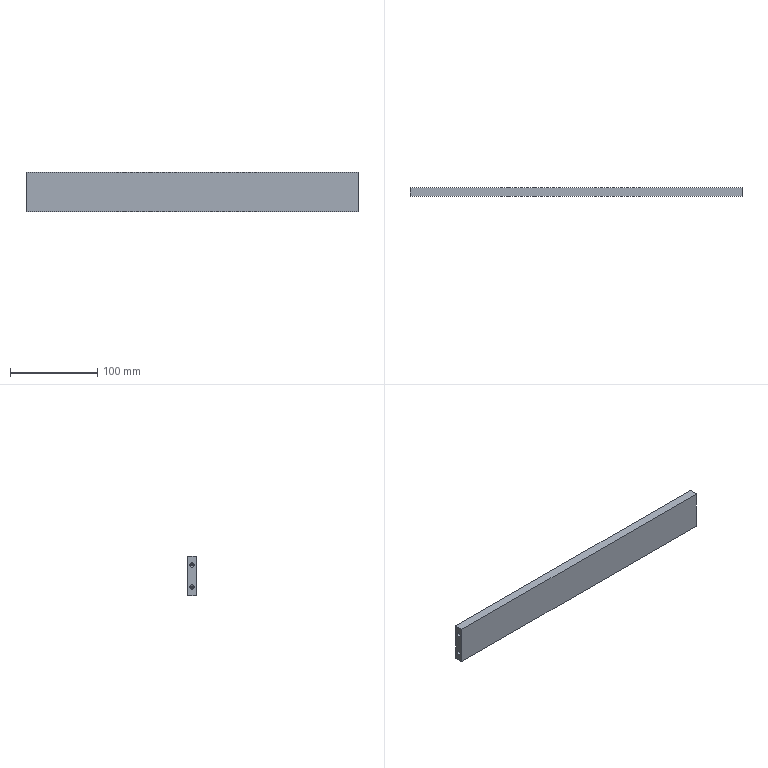Component | SolidWorks | 01-08MarkingMachineDrumConnectingPlate2-1 | 1 solid | 22 faces | box 380 x 10 x 45 mm | volume 169783 mm3 | cylinder 8 | cone 8 | plane 6 | commonest cylinder face diameters 5 x8 | material A3 Steel
build123d program:
from build123d import *

# Parameters (mm, degrees)
SKETCH1_W                  = 380
SKETCH1_H                  = 45
BOSS_EXTRUDE1_DEPTH        = 5
M6_TAPPED_HOLE1_AT_2_COUNT = 2
M6_TAPPED_HOLE1_AT_2_PITCH = 25


with BuildPart() as part:
    # Sketch1 → Boss-Extrude1 (new, symmetric)
    with BuildSketch(Plane.XY):
        Rectangle(SKETCH1_W, SKETCH1_H)
    extrude(amount=BOSS_EXTRUDE1_DEPTH, both=True)

    # Sketch4 → M6 Tapped Hole1 (revolve, cut)
    with BuildSketch(Plane(origin=(190, 12.5, 0), x_dir=(0, 0, -1), z_dir=(0, 1, 0))):
        Polygon((0, 0), (0, 16.502), (2.5, 15), (2.5, 0), align=None)
    m6_tapped_hole1 = revolve(axis=Axis((196.35, 12.5, 0), (-1, 0, 0)), mode=Mode.SUBTRACT)

    # M6 Tapped Hole1 at 2: M6 Tapped Hole1 ×2
    with Locations(*[(0, -i * M6_TAPPED_HOLE1_AT_2_PITCH, 0) for i in range(1, M6_TAPPED_HOLE1_AT_2_COUNT)]):
        add(m6_tapped_hole1, mode=Mode.SUBTRACT)

    # Mirror1: M6 Tapped Hole1 across plane
    add(m6_tapped_hole1.mirror(Plane(origin=(0, 0, 0), x_dir=(0, 0, 1), z_dir=(1, 0, 0))), mode=Mode.SUBTRACT)

    # Mirror1 copy 1 sketch → Mirror1 copy 1 (revolve, cut)
    with BuildSketch(Plane(origin=(-190, -12.5, 0), x_dir=(0, 0, -1), z_dir=(0, 1, 0))):
        Polygon((0, 0), (0, -16.502), (2.5, -15), (2.5, 0), align=None)
    revolve(axis=Axis((-196.35, -12.5, 0), (-1, 0, 0)), mode=Mode.SUBTRACT)


solid = part.part

# Placed as in the assembly
solid = solid.moved(Location((-256.91, 2.41, -167.5), (90, 0, 0)))
STEP:
#1=COLOUR_RGB('',0.7922,0.8196,0.9333);
#2=FILL_AREA_STYLE_COLOUR('',#1);
#3=FILL_AREA_STYLE('',(#2));
#4=SURFACE_STYLE_FILL_AREA(#3);
#5=SURFACE_SIDE_STYLE('',(#4));
#6=SURFACE_STYLE_USAGE(.BOTH.,#5);
#7=PRESENTATION_STYLE_ASSIGNMENT((#6));
#8=CARTESIAN_POINT('',(-17.004,0.1933,-6.102));
#9=VERTEX_POINT('',#8);
#10=CARTESIAN_POINT('',(-17.004,-0.003525,-6.102));
#11=VERTEX_POINT('',#10);
#12=CARTESIAN_POINT('',(-17.004,0.0949,-6.102));
#13=DIRECTION('',(-1.,0.,0.));
#14=DIRECTION('',(0.,-1.,0.));
#15=AXIS2_PLACEMENT_3D('',#12,#13,#14);
#16=CIRCLE('',#15,0.09843);
#17=EDGE_CURVE('',#9,#11,#16,.T.);
#18=ORIENTED_EDGE('',*,*,#17,.F.);
#19=CARTESIAN_POINT('',(-17.595,0.1933,-6.102));
#20=VERTEX_POINT('',#19);
#21=CARTESIAN_POINT('',(-17.595,0.1933,-6.102));
#22=DIRECTION('',(-1.,0.,0.));
#23=VECTOR('',#22,39.37);
#24=LINE('',#21,#23);
#25=EDGE_CURVE('',#9,#20,#24,.T.);
#26=ORIENTED_EDGE('',*,*,#25,.T.);
#27=CARTESIAN_POINT('',(-17.595,-0.003525,-6.102));
#28=VERTEX_POINT('',#27);
#29=CARTESIAN_POINT('',(-17.595,0.0949,-6.102));
#30=DIRECTION('',(-1.,0.,0.));
#31=DIRECTION('',(0.,-1.,0.));
#32=AXIS2_PLACEMENT_3D('',#29,#30,#31);
#33=CIRCLE('',#32,0.09843);
#34=EDGE_CURVE('',#20,#28,#33,.T.);
#35=ORIENTED_EDGE('',*,*,#34,.T.);
#36=CARTESIAN_POINT('',(-17.595,-0.003525,-6.102));
#37=DIRECTION('',(-1.,0.,0.));
#38=VECTOR('',#37,39.37);
#39=LINE('',#36,#38);
#40=EDGE_CURVE('',#11,#28,#39,.T.);
#41=ORIENTED_EDGE('',*,*,#40,.F.);
#42=EDGE_LOOP('',(#18,#26,#35,#41));
#43=FACE_OUTER_BOUND('',#42,.T.);
#44=CARTESIAN_POINT('',(-17.595,0.0949,-6.102));
#45=DIRECTION('',(-1.,0.,0.));
#46=DIRECTION('',(0.,-1.,0.));
#47=AXIS2_PLACEMENT_3D('',#44,#45,#46);
#48=CYLINDRICAL_SURFACE('',#47,0.09843);
#49=ADVANCED_FACE('',(#43),#48,.F.);
#50=CARTESIAN_POINT('',(-16.945,0.0949,-6.102));
#51=VERTEX_POINT('',#50);
#52=CARTESIAN_POINT('',(-17.004,-0.003525,-6.102));
#53=DIRECTION('',(-0.515,-0.8572,-0.));
#54=VECTOR('',#53,39.37);
#55=LINE('',#52,#54);
#56=EDGE_CURVE('',#51,#11,#55,.T.);
#57=ORIENTED_EDGE('',*,*,#56,.F.);
#58=CARTESIAN_POINT('',(-17.004,0.1933,-6.102));
#59=DIRECTION('',(-0.515,0.8572,0.));
#60=VECTOR('',#59,39.37);
#61=LINE('',#58,#60);
#62=EDGE_CURVE('',#51,#9,#61,.T.);
#63=ORIENTED_EDGE('',*,*,#62,.T.);
#64=ORIENTED_EDGE('',*,*,#17,.T.);
#65=EDGE_LOOP('',(#57,#63,#64));
#66=FACE_OUTER_BOUND('',#65,.T.);
#67=CARTESIAN_POINT('',(-17.004,0.0949,-6.102));
#68=DIRECTION('',(-1.,0.,0.));
#69=DIRECTION('',(0.,-1.,0.));
#70=AXIS2_PLACEMENT_3D('',#67,#68,#69);
#71=CONICAL_SURFACE('',#70,0.09843,1.03);
#72=ADVANCED_FACE('',(#66),#71,.F.);
#73=CARTESIAN_POINT('',(-17.004,0.1933,-7.087));
#74=VERTEX_POINT('',#73);
#75=CARTESIAN_POINT('',(-17.004,-0.003525,-7.087));
#76=VERTEX_POINT('',#75);
#77=CARTESIAN_POINT('',(-17.004,0.0949,-7.087));
#78=DIRECTION('',(-1.,0.,0.));
#79=DIRECTION('',(0.,-1.,0.));
#80=AXIS2_PLACEMENT_3D('',#77,#78,#79);
#81=CIRCLE('',#80,0.09843);
#82=EDGE_CURVE('',#74,#76,#81,.T.);
#83=ORIENTED_EDGE('',*,*,#82,.F.);
#84=CARTESIAN_POINT('',(-17.595,0.1933,-7.087));
#85=VERTEX_POINT('',#84);
#86=CARTESIAN_POINT('',(-17.595,0.1933,-7.087));
#87=DIRECTION('',(-1.,0.,0.));
#88=VECTOR('',#87,39.37);
#89=LINE('',#86,#88);
#90=EDGE_CURVE('',#74,#85,#89,.T.);
#91=ORIENTED_EDGE('',*,*,#90,.T.);
#92=CARTESIAN_POINT('',(-17.595,-0.003525,-7.087));
#93=VERTEX_POINT('',#92);
#94=CARTESIAN_POINT('',(-17.595,0.0949,-7.087));
#95=DIRECTION('',(-1.,0.,0.));
#96=DIRECTION('',(0.,-1.,0.));
#97=AXIS2_PLACEMENT_3D('',#94,#95,#96);
#98=CIRCLE('',#97,0.09843);
#99=EDGE_CURVE('',#85,#93,#98,.T.);
#100=ORIENTED_EDGE('',*,*,#99,.T.);
#101=CARTESIAN_POINT('',(-17.595,-0.003525,-7.087));
#102=DIRECTION('',(-1.,0.,0.));
#103=VECTOR('',#102,39.37);
#104=LINE('',#101,#103);
#105=EDGE_CURVE('',#76,#93,#104,.T.);
#106=ORIENTED_EDGE('',*,*,#105,.F.);
#107=EDGE_LOOP('',(#83,#91,#100,#106));
#108=FACE_OUTER_BOUND('',#107,.T.);
#109=CARTESIAN_POINT('',(-17.595,0.0949,-7.087));
#110=DIRECTION('',(-1.,0.,0.));
#111=DIRECTION('',(0.,-1.,0.));
#112=AXIS2_PLACEMENT_3D('',#109,#110,#111);
#113=CYLINDRICAL_SURFACE('',#112,0.09843);
#114=ADVANCED_FACE('',(#108),#113,.F.);
#115=CARTESIAN_POINT('',(-16.945,0.0949,-7.087));
#116=VERTEX_POINT('',#115);
#117=CARTESIAN_POINT('',(-17.004,-0.003525,-7.087));
#118=DIRECTION('',(-0.515,-0.8572,-0.));
#119=VECTOR('',#118,39.37);
#120=LINE('',#117,#119);
#121=EDGE_CURVE('',#116,#76,#120,.T.);
#122=ORIENTED_EDGE('',*,*,#121,.F.);
#123=CARTESIAN_POINT('',(-17.004,0.1933,-7.087));
#124=DIRECTION('',(-0.515,0.8572,0.));
#125=VECTOR('',#124,39.37);
#126=LINE('',#123,#125);
#127=EDGE_CURVE('',#116,#74,#126,.T.);
#128=ORIENTED_EDGE('',*,*,#127,.T.);
#129=ORIENTED_EDGE('',*,*,#82,.T.);
#130=EDGE_LOOP('',(#122,#128,#129));
#131=FACE_OUTER_BOUND('',#130,.T.);
#132=CARTESIAN_POINT('',(-17.004,0.0949,-7.087));
#133=DIRECTION('',(-1.,0.,0.));
#134=DIRECTION('',(0.,-1.,0.));
#135=AXIS2_PLACEMENT_3D('',#132,#133,#134);
#136=CONICAL_SURFACE('',#135,0.09843,1.03);
#137=ADVANCED_FACE('',(#131),#136,.F.);
#138=CARTESIAN_POINT('',(-3.225,-0.003525,-6.102));
#139=VERTEX_POINT('',#138);
#140=CARTESIAN_POINT('',(-3.225,0.1933,-6.102));
#141=VERTEX_POINT('',#140);
#142=CARTESIAN_POINT('',(-3.225,0.0949,-6.102));
#143=DIRECTION('',(1.,-0.,-0.));
#144=DIRECTION('',(0.,1.,0.));
#145=AXIS2_PLACEMENT_3D('',#142,#143,#144);
#146=CIRCLE('',#145,0.09843);
#147=EDGE_CURVE('',#139,#141,#146,.T.);
#148=ORIENTED_EDGE('',*,*,#147,.F.);
#149=CARTESIAN_POINT('',(-2.634,-0.003525,-6.102));
#150=VERTEX_POINT('',#149);
#151=CARTESIAN_POINT('',(-2.634,-0.003525,-6.102));
#152=DIRECTION('',(1.,-0.,-0.));
#153=VECTOR('',#152,39.37);
#154=LINE('',#151,#153);
#155=EDGE_CURVE('',#139,#150,#154,.T.);
#156=ORIENTED_EDGE('',*,*,#155,.T.);
#157=CARTESIAN_POINT('',(-2.634,0.1933,-6.102));
#158=VERTEX_POINT('',#157);
#159=CARTESIAN_POINT('',(-2.634,0.0949,-6.102));
#160=DIRECTION('',(1.,-0.,-0.));
#161=DIRECTION('',(0.,1.,0.));
#162=AXIS2_PLACEMENT_3D('',#159,#160,#161);
#163=CIRCLE('',#162,0.09843);
#164=EDGE_CURVE('',#150,#158,#163,.T.);
#165=ORIENTED_EDGE('',*,*,#164,.T.);
#166=CARTESIAN_POINT('',(-2.634,0.1933,-6.102));
#167=DIRECTION('',(1.,-0.,-0.));
#168=VECTOR('',#167,39.37);
#169=LINE('',#166,#168);
#170=EDGE_CURVE('',#141,#158,#169,.T.);
#171=ORIENTED_EDGE('',*,*,#170,.F.);
#172=EDGE_LOOP('',(#148,#156,#165,#171));
#173=FACE_OUTER_BOUND('',#172,.T.);
#174=CARTESIAN_POINT('',(-2.634,0.0949,-6.102));
#175=DIRECTION('',(1.,-0.,-0.));
#176=DIRECTION('',(0.,1.,0.));
#177=AXIS2_PLACEMENT_3D('',#174,#175,#176);
#178=CYLINDRICAL_SURFACE('',#177,0.09843);
#179=ADVANCED_FACE('',(#173),#178,.F.);
#180=CARTESIAN_POINT('',(-3.284,0.0949,-6.102));
#181=VERTEX_POINT('',#180);
#182=CARTESIAN_POINT('',(-3.225,0.1933,-6.102));
#183=DIRECTION('',(0.515,0.8572,0.));
#184=VECTOR('',#183,39.37);
#185=LINE('',#182,#184);
#186=EDGE_CURVE('',#181,#141,#185,.T.);
#187=ORIENTED_EDGE('',*,*,#186,.F.);
#188=CARTESIAN_POINT('',(-3.225,-0.003525,-6.102));
#189=DIRECTION('',(0.515,-0.8572,0.));
#190=VECTOR('',#189,39.37);
#191=LINE('',#188,#190);
#192=EDGE_CURVE('',#181,#139,#191,.T.);
#193=ORIENTED_EDGE('',*,*,#192,.T.);
#194=ORIENTED_EDGE('',*,*,#147,.T.);
#195=EDGE_LOOP('',(#187,#193,#194));
#196=FACE_OUTER_BOUND('',#195,.T.);
#197=CARTESIAN_POINT('',(-3.225,0.0949,-6.102));
#198=DIRECTION('',(1.,-0.,-0.));
#199=DIRECTION('',(0.,1.,0.));
#200=AXIS2_PLACEMENT_3D('',#197,#198,#199);
#201=CONICAL_SURFACE('',#200,0.09843,1.03);
#202=ADVANCED_FACE('',(#196),#201,.F.);
#203=CARTESIAN_POINT('',(-3.225,-0.003525,-7.087));
#204=VERTEX_POINT('',#203);
#205=CARTESIAN_POINT('',(-3.225,0.1933,-7.087));
#206=VERTEX_POINT('',#205);
#207=CARTESIAN_POINT('',(-3.225,0.0949,-7.087));
#208=DIRECTION('',(1.,-0.,-0.));
#209=DIRECTION('',(0.,1.,0.));
#210=AXIS2_PLACEMENT_3D('',#207,#208,#209);
#211=CIRCLE('',#210,0.09843);
#212=EDGE_CURVE('',#204,#206,#211,.T.);
#213=ORIENTED_EDGE('',*,*,#212,.F.);
#214=CARTESIAN_POINT('',(-2.634,-0.003525,-7.087));
#215=VERTEX_POINT('',#214);
#216=CARTESIAN_POINT('',(-2.634,-0.003525,-7.087));
#217=DIRECTION('',(1.,-0.,-0.));
#218=VECTOR('',#217,39.37);
#219=LINE('',#216,#218);
#220=EDGE_CURVE('',#204,#215,#219,.T.);
#221=ORIENTED_EDGE('',*,*,#220,.T.);
#222=CARTESIAN_POINT('',(-2.634,0.1933,-7.087));
#223=VERTEX_POINT('',#222);
#224=CARTESIAN_POINT('',(-2.634,0.0949,-7.087));
#225=DIRECTION('',(1.,-0.,-0.));
#226=DIRECTION('',(0.,1.,0.));
#227=AXIS2_PLACEMENT_3D('',#224,#225,#226);
#228=CIRCLE('',#227,0.09843);
#229=EDGE_CURVE('',#215,#223,#228,.T.);
#230=ORIENTED_EDGE('',*,*,#229,.T.);
#231=CARTESIAN_POINT('',(-2.634,0.1933,-7.087));
#232=DIRECTION('',(1.,-0.,-0.));
#233=VECTOR('',#232,39.37);
#234=LINE('',#231,#233);
#235=EDGE_CURVE('',#206,#223,#234,.T.);
#236=ORIENTED_EDGE('',*,*,#235,.F.);
#237=EDGE_LOOP('',(#213,#221,#230,#236));
#238=FACE_OUTER_BOUND('',#237,.T.);
#239=CARTESIAN_POINT('',(-2.634,0.0949,-7.087));
#240=DIRECTION('',(1.,-0.,-0.));
#241=DIRECTION('',(0.,1.,0.));
#242=AXIS2_PLACEMENT_3D('',#239,#240,#241);
#243=CYLINDRICAL_SURFACE('',#242,0.09843);
#244=ADVANCED_FACE('',(#238),#243,.F.);
#245=CARTESIAN_POINT('',(-3.284,0.0949,-7.087));
#246=VERTEX_POINT('',#245);
#247=CARTESIAN_POINT('',(-3.225,0.1933,-7.087));
#248=DIRECTION('',(0.515,0.8572,0.));
#249=VECTOR('',#248,39.37);
#250=LINE('',#247,#249);
#251=EDGE_CURVE('',#246,#206,#250,.T.);
#252=ORIENTED_EDGE('',*,*,#251,.F.);
#253=CARTESIAN_POINT('',(-3.225,-0.003525,-7.087));
#254=DIRECTION('',(0.515,-0.8572,0.));
#255=VECTOR('',#254,39.37);
#256=LINE('',#253,#255);
#257=EDGE_CURVE('',#246,#204,#256,.T.);
#258=ORIENTED_EDGE('',*,*,#257,.T.);
#259=ORIENTED_EDGE('',*,*,#212,.T.);
#260=EDGE_LOOP('',(#252,#258,#259));
#261=FACE_OUTER_BOUND('',#260,.T.);
#262=CARTESIAN_POINT('',(-3.225,0.0949,-7.087));
#263=DIRECTION('',(1.,-0.,-0.));
#264=DIRECTION('',(0.,1.,0.));
#265=AXIS2_PLACEMENT_3D('',#262,#263,#264);
#266=CONICAL_SURFACE('',#265,0.09843,1.03);
#267=ADVANCED_FACE('',(#261),#266,.F.);
#268=CARTESIAN_POINT('',(-17.595,0.0949,-7.087));
#269=DIRECTION('',(-1.,0.,0.));
#270=DIRECTION('',(0.,-1.,0.));
#271=AXIS2_PLACEMENT_3D('',#268,#269,#270);
#272=CIRCLE('',#271,0.09843);
#273=EDGE_CURVE('',#93,#85,#272,.T.);
#274=ORIENTED_EDGE('',*,*,#273,.F.);
#275=ORIENTED_EDGE('',*,*,#99,.F.);
#276=EDGE_LOOP('',(#274,#275));
#277=FACE_BOUND('',#276,.T.);
#278=CARTESIAN_POINT('',(-17.595,0.2918,-5.709));
#279=VERTEX_POINT('',#278);
#280=CARTESIAN_POINT('',(-17.595,0.2918,-7.48));
#281=VERTEX_POINT('',#280);
#282=CARTESIAN_POINT('',(-17.595,0.2918,-7.48));
#283=DIRECTION('',(-0.,0.,-1.));
#284=VECTOR('',#283,39.37);
#285=LINE('',#282,#284);
#286=EDGE_CURVE('',#279,#281,#285,.T.);
#287=ORIENTED_EDGE('',*,*,#286,.T.);
#288=CARTESIAN_POINT('',(-17.595,-0.102,-7.48));
#289=VERTEX_POINT('',#288);
#290=CARTESIAN_POINT('',(-17.595,-0.102,-7.48));
#291=DIRECTION('',(0.,1.,0.));
#292=VECTOR('',#291,39.37);
#293=LINE('',#290,#292);
#294=EDGE_CURVE('',#289,#281,#293,.T.);
#295=ORIENTED_EDGE('',*,*,#294,.F.);
#296=CARTESIAN_POINT('',(-17.595,-0.102,-5.709));
#297=VERTEX_POINT('',#296);
#298=CARTESIAN_POINT('',(-17.595,-0.102,-7.48));
#299=DIRECTION('',(-0.,0.,-1.));
#300=VECTOR('',#299,39.37);
#301=LINE('',#298,#300);
#302=EDGE_CURVE('',#297,#289,#301,.T.);
#303=ORIENTED_EDGE('',*,*,#302,.F.);
#304=CARTESIAN_POINT('',(-17.595,-0.102,-5.709));
#305=DIRECTION('',(0.,1.,0.));
#306=VECTOR('',#305,39.37);
#307=LINE('',#304,#306);
#308=EDGE_CURVE('',#297,#279,#307,.T.);
#309=ORIENTED_EDGE('',*,*,#308,.T.);
#310=EDGE_LOOP('',(#287,#295,#303,#309));
#311=FACE_OUTER_BOUND('',#310,.T.);
#312=CARTESIAN_POINT('',(-17.595,0.0949,-6.102));
#313=DIRECTION('',(-1.,0.,0.));
#314=DIRECTION('',(0.,-1.,0.));
#315=AXIS2_PLACEMENT_3D('',#312,#313,#314);
#316=CIRCLE('',#315,0.09843);
#317=EDGE_CURVE('',#28,#20,#316,.T.);
#318=ORIENTED_EDGE('',*,*,#317,.F.);
#319=ORIENTED_EDGE('',*,*,#34,.F.);
#320=EDGE_LOOP('',(#318,#319));
#321=FACE_BOUND('',#320,.T.);
#322=CARTESIAN_POINT('',(-17.595,-0.102,-7.48));
#323=DIRECTION('',(1.,-0.,-0.));
#324=DIRECTION('',(0.,1.,0.));
#325=AXIS2_PLACEMENT_3D('',#322,#323,#324);
#326=PLANE('',#325);
#327=ADVANCED_FACE('',(#277,#311,#321),#326,.F.);
#328=CARTESIAN_POINT('',(-2.634,0.0949,-7.087));
#329=DIRECTION('',(1.,-0.,-0.));
#330=DIRECTION('',(0.,1.,0.));
#331=AXIS2_PLACEMENT_3D('',#328,#329,#330);
#332=CIRCLE('',#331,0.09843);
#333=EDGE_CURVE('',#223,#215,#332,.T.);
#334=ORIENTED_EDGE('',*,*,#333,.F.);
#335=ORIENTED_EDGE('',*,*,#229,.F.);
#336=EDGE_LOOP('',(#334,#335));
#337=FACE_BOUND('',#336,.T.);
#338=CARTESIAN_POINT('',(-2.634,0.2918,-7.48));
#339=VERTEX_POINT('',#338);
#340=CARTESIAN_POINT('',(-2.634,0.2918,-5.709));
#341=VERTEX_POINT('',#340);
#342=CARTESIAN_POINT('',(-2.634,0.2918,-7.48));
#343=DIRECTION('',(0.,-0.,1.));
#344=VECTOR('',#343,39.37);
#345=LINE('',#342,#344);
#346=EDGE_CURVE('',#339,#341,#345,.T.);
#347=ORIENTED_EDGE('',*,*,#346,.T.);
#348=CARTESIAN_POINT('',(-2.634,-0.102,-5.709));
#349=VERTEX_POINT('',#348);
#350=CARTESIAN_POINT('',(-2.634,-0.102,-5.709));
#351=DIRECTION('',(0.,1.,0.));
#352=VECTOR('',#351,39.37);
#353=LINE('',#350,#352);
#354=EDGE_CURVE('',#349,#341,#353,.T.);
#355=ORIENTED_EDGE('',*,*,#354,.F.);
#356=CARTESIAN_POINT('',(-2.634,-0.102,-7.48));
#357=VERTEX_POINT('',#356);
#358=CARTESIAN_POINT('',(-2.634,-0.102,-7.48));
#359=DIRECTION('',(0.,-0.,1.));
#360=VECTOR('',#359,39.37);
#361=LINE('',#358,#360);
#362=EDGE_CURVE('',#357,#349,#361,.T.);
#363=ORIENTED_EDGE('',*,*,#362,.F.);
#364=CARTESIAN_POINT('',(-2.634,-0.102,-7.48));
#365=DIRECTION('',(0.,1.,0.));
#366=VECTOR('',#365,39.37);
#367=LINE('',#364,#366);
#368=EDGE_CURVE('',#357,#339,#367,.T.);
#369=ORIENTED_EDGE('',*,*,#368,.T.);
#370=EDGE_LOOP('',(#347,#355,#363,#369));
#371=FACE_OUTER_BOUND('',#370,.T.);
#372=CARTESIAN_POINT('',(-2.634,0.0949,-6.102));
#373=DIRECTION('',(1.,-0.,-0.));
#374=DIRECTION('',(0.,1.,0.));
#375=AXIS2_PLACEMENT_3D('',#372,#373,#374);
#376=CIRCLE('',#375,0.09843);
#377=EDGE_CURVE('',#158,#150,#376,.T.);
#378=ORIENTED_EDGE('',*,*,#377,.F.);
#379=ORIENTED_EDGE('',*,*,#164,.F.);
#380=EDGE_LOOP('',(#378,#379));
#381=FACE_BOUND('',#380,.T.);
#382=CARTESIAN_POINT('',(-2.634,-0.102,-7.48));
#383=DIRECTION('',(-1.,0.,0.));
#384=DIRECTION('',(-0.,-1.,-0.));
#385=AXIS2_PLACEMENT_3D('',#382,#383,#384);
#386=PLANE('',#385);
#387=ADVANCED_FACE('',(#337,#371,#381),#386,.F.);
#388=CARTESIAN_POINT('',(-17.595,0.2918,-5.709));
#389=DIRECTION('',(-1.,0.,0.));
#390=VECTOR('',#389,39.37);
#391=LINE('',#388,#390);
#392=EDGE_CURVE('',#341,#279,#391,.T.);
#393=ORIENTED_EDGE('',*,*,#392,.T.);
#394=ORIENTED_EDGE('',*,*,#308,.F.);
#395=CARTESIAN_POINT('',(-17.595,-0.102,-5.709));
#396=DIRECTION('',(-1.,0.,0.));
#397=VECTOR('',#396,39.37);
#398=LINE('',#395,#397);
#399=EDGE_CURVE('',#349,#297,#398,.T.);
#400=ORIENTED_EDGE('',*,*,#399,.F.);
#401=ORIENTED_EDGE('',*,*,#354,.T.);
#402=EDGE_LOOP('',(#393,#394,#400,#401));
#403=FACE_OUTER_BOUND('',#402,.T.);
#404=CARTESIAN_POINT('',(-17.595,-0.102,-5.709));
#405=DIRECTION('',(-0.,0.,-1.));
#406=DIRECTION('',(0.,1.,0.));
#407=AXIS2_PLACEMENT_3D('',#404,#405,#406);
#408=PLANE('',#407);
#409=ADVANCED_FACE('',(#403),#408,.F.);
#410=CARTESIAN_POINT('',(-17.595,0.2918,-7.48));
#411=DIRECTION('',(1.,-0.,-0.));
#412=VECTOR('',#411,39.37);
#413=LINE('',#410,#412);
#414=EDGE_CURVE('',#281,#339,#413,.T.);
#415=ORIENTED_EDGE('',*,*,#414,.T.);
#416=ORIENTED_EDGE('',*,*,#368,.F.);
#417=CARTESIAN_POINT('',(-17.595,-0.102,-7.48));
#418=DIRECTION('',(1.,-0.,-0.));
#419=VECTOR('',#418,39.37);
#420=LINE('',#417,#419);
#421=EDGE_CURVE('',#289,#357,#420,.T.);
#422=ORIENTED_EDGE('',*,*,#421,.F.);
#423=ORIENTED_EDGE('',*,*,#294,.T.);
#424=EDGE_LOOP('',(#415,#416,#422,#423));
#425=FACE_OUTER_BOUND('',#424,.T.);
#426=CARTESIAN_POINT('',(-17.595,-0.102,-7.48));
#427=DIRECTION('',(0.,-0.,1.));
#428=DIRECTION('',(-0.,-1.,-0.));
#429=AXIS2_PLACEMENT_3D('',#426,#427,#428);
#430=PLANE('',#429);
#431=ADVANCED_FACE('',(#425),#430,.F.);
#432=ORIENTED_EDGE('',*,*,#362,.T.);
#433=ORIENTED_EDGE('',*,*,#399,.T.);
#434=ORIENTED_EDGE('',*,*,#302,.T.);
#435=ORIENTED_EDGE('',*,*,#421,.T.);
#436=EDGE_LOOP('',(#432,#433,#434,#435));
#437=FACE_OUTER_BOUND('',#436,.T.);
#438=CARTESIAN_POINT('',(-10.115,-0.102,-6.594));
#439=DIRECTION('',(0.,1.,0.));
#440=DIRECTION('',(-1.,0.,0.));
#441=AXIS2_PLACEMENT_3D('',#438,#439,#440);
#442=PLANE('',#441);
#443=ADVANCED_FACE('',(#437),#442,.F.);
#444=ORIENTED_EDGE('',*,*,#346,.F.);
#445=ORIENTED_EDGE('',*,*,#414,.F.);
#446=ORIENTED_EDGE('',*,*,#286,.F.);
#447=ORIENTED_EDGE('',*,*,#392,.F.);
#448=EDGE_LOOP('',(#444,#445,#446,#447));
#449=FACE_OUTER_BOUND('',#448,.T.);
#450=CARTESIAN_POINT('',(-10.115,0.2918,-6.594));
#451=DIRECTION('',(0.,1.,0.));
#452=DIRECTION('',(-1.,0.,0.));
#453=AXIS2_PLACEMENT_3D('',#450,#451,#452);
#454=PLANE('',#453);
#455=ADVANCED_FACE('',(#449),#454,.T.);
#456=ORIENTED_EDGE('',*,*,#257,.F.);
#457=ORIENTED_EDGE('',*,*,#251,.T.);
#458=CARTESIAN_POINT('',(-3.225,0.0949,-7.087));
#459=DIRECTION('',(1.,-0.,-0.));
#460=DIRECTION('',(0.,1.,0.));
#461=AXIS2_PLACEMENT_3D('',#458,#459,#460);
#462=CIRCLE('',#461,0.09843);
#463=EDGE_CURVE('',#206,#204,#462,.T.);
#464=ORIENTED_EDGE('',*,*,#463,.T.);
#465=EDGE_LOOP('',(#456,#457,#464));
#466=FACE_OUTER_BOUND('',#465,.T.);
#467=CARTESIAN_POINT('',(-3.225,0.0949,-7.087));
#468=DIRECTION('',(1.,-0.,-0.));
#469=DIRECTION('',(0.,1.,0.));
#470=AXIS2_PLACEMENT_3D('',#467,#468,#469);
#471=CONICAL_SURFACE('',#470,0.09843,1.03);
#472=ADVANCED_FACE('',(#466),#471,.F.);
#473=ORIENTED_EDGE('',*,*,#220,.F.);
#474=ORIENTED_EDGE('',*,*,#463,.F.);
#475=ORIENTED_EDGE('',*,*,#235,.T.);
#476=ORIENTED_EDGE('',*,*,#333,.T.);
#477=EDGE_LOOP('',(#473,#474,#475,#476));
#478=FACE_OUTER_BOUND('',#477,.T.);
#479=CARTESIAN_POINT('',(-2.634,0.0949,-7.087));
#480=DIRECTION('',(1.,-0.,-0.));
#481=DIRECTION('',(0.,1.,0.));
#482=AXIS2_PLACEMENT_3D('',#479,#480,#481);
#483=CYLINDRICAL_SURFACE('',#482,0.09843);
#484=ADVANCED_FACE('',(#478),#483,.F.);
#485=ORIENTED_EDGE('',*,*,#192,.F.);
#486=ORIENTED_EDGE('',*,*,#186,.T.);
#487=CARTESIAN_POINT('',(-3.225,0.0949,-6.102));
#488=DIRECTION('',(1.,-0.,-0.));
#489=DIRECTION('',(0.,1.,0.));
#490=AXIS2_PLACEMENT_3D('',#487,#488,#489);
#491=CIRCLE('',#490,0.09843);
#492=EDGE_CURVE('',#141,#139,#491,.T.);
#493=ORIENTED_EDGE('',*,*,#492,.T.);
#494=EDGE_LOOP('',(#485,#486,#493));
#495=FACE_OUTER_BOUND('',#494,.T.);
#496=CARTESIAN_POINT('',(-3.225,0.0949,-6.102));
#497=DIRECTION('',(1.,-0.,-0.));
#498=DIRECTION('',(0.,1.,0.));
#499=AXIS2_PLACEMENT_3D('',#496,#497,#498);
#500=CONICAL_SURFACE('',#499,0.09843,1.03);
#501=ADVANCED_FACE('',(#495),#500,.F.);
#502=ORIENTED_EDGE('',*,*,#155,.F.);
#503=ORIENTED_EDGE('',*,*,#492,.F.);
#504=ORIENTED_EDGE('',*,*,#170,.T.);
#505=ORIENTED_EDGE('',*,*,#377,.T.);
#506=EDGE_LOOP('',(#502,#503,#504,#505));
#507=FACE_OUTER_BOUND('',#506,.T.);
#508=CARTESIAN_POINT('',(-2.634,0.0949,-6.102));
#509=DIRECTION('',(1.,-0.,-0.));
#510=DIRECTION('',(0.,1.,0.));
#511=AXIS2_PLACEMENT_3D('',#508,#509,#510);
#512=CYLINDRICAL_SURFACE('',#511,0.09843);
#513=ADVANCED_FACE('',(#507),#512,.F.);
#514=ORIENTED_EDGE('',*,*,#127,.F.);
#515=ORIENTED_EDGE('',*,*,#121,.T.);
#516=CARTESIAN_POINT('',(-17.004,0.0949,-7.087));
#517=DIRECTION('',(-1.,0.,0.));
#518=DIRECTION('',(0.,-1.,0.));
#519=AXIS2_PLACEMENT_3D('',#516,#517,#518);
#520=CIRCLE('',#519,0.09843);
#521=EDGE_CURVE('',#76,#74,#520,.T.);
#522=ORIENTED_EDGE('',*,*,#521,.T.);
#523=EDGE_LOOP('',(#514,#515,#522));
#524=FACE_OUTER_BOUND('',#523,.T.);
#525=CARTESIAN_POINT('',(-17.004,0.0949,-7.087));
#526=DIRECTION('',(-1.,0.,0.));
#527=DIRECTION('',(0.,-1.,0.));
#528=AXIS2_PLACEMENT_3D('',#525,#526,#527);
#529=CONICAL_SURFACE('',#528,0.09843,1.03);
#530=ADVANCED_FACE('',(#524),#529,.F.);
#531=ORIENTED_EDGE('',*,*,#90,.F.);
#532=ORIENTED_EDGE('',*,*,#521,.F.);
#533=ORIENTED_EDGE('',*,*,#105,.T.);
#534=ORIENTED_EDGE('',*,*,#273,.T.);
#535=EDGE_LOOP('',(#531,#532,#533,#534));
#536=FACE_OUTER_BOUND('',#535,.T.);
#537=CARTESIAN_POINT('',(-17.595,0.0949,-7.087));
#538=DIRECTION('',(-1.,0.,0.));
#539=DIRECTION('',(0.,-1.,0.));
#540=AXIS2_PLACEMENT_3D('',#537,#538,#539);
#541=CYLINDRICAL_SURFACE('',#540,0.09843);
#542=ADVANCED_FACE('',(#536),#541,.F.);
#543=ORIENTED_EDGE('',*,*,#62,.F.);
#544=ORIENTED_EDGE('',*,*,#56,.T.);
#545=CARTESIAN_POINT('',(-17.004,0.0949,-6.102));
#546=DIRECTION('',(-1.,0.,0.));
#547=DIRECTION('',(0.,-1.,0.));
#548=AXIS2_PLACEMENT_3D('',#545,#546,#547);
#549=CIRCLE('',#548,0.09843);
#550=EDGE_CURVE('',#11,#9,#549,.T.);
#551=ORIENTED_EDGE('',*,*,#550,.T.);
#552=EDGE_LOOP('',(#543,#544,#551));
#553=FACE_OUTER_BOUND('',#552,.T.);
#554=CARTESIAN_POINT('',(-17.004,0.0949,-6.102));
#555=DIRECTION('',(-1.,0.,0.));
#556=DIRECTION('',(0.,-1.,0.));
#557=AXIS2_PLACEMENT_3D('',#554,#555,#556);
#558=CONICAL_SURFACE('',#557,0.09843,1.03);
#559=ADVANCED_FACE('',(#553),#558,.F.);
#560=ORIENTED_EDGE('',*,*,#25,.F.);
#561=ORIENTED_EDGE('',*,*,#550,.F.);
#562=ORIENTED_EDGE('',*,*,#40,.T.);
#563=ORIENTED_EDGE('',*,*,#317,.T.);
#564=EDGE_LOOP('',(#560,#561,#562,#563));
#565=FACE_OUTER_BOUND('',#564,.T.);
#566=CARTESIAN_POINT('',(-17.595,0.0949,-6.102));
#567=DIRECTION('',(-1.,0.,0.));
#568=DIRECTION('',(0.,-1.,0.));
#569=AXIS2_PLACEMENT_3D('',#566,#567,#568);
#570=CYLINDRICAL_SURFACE('',#569,0.09843);
#571=ADVANCED_FACE('',(#565),#570,.F.);
#572=CLOSED_SHELL('',(#49,#72,#114,#137,#179,#202,#244,#267,#327,#387,#409,#431,#443,#455,#472,#484,#501,#513,#530,#542,#559,#571));
#573=MANIFOLD_SOLID_BREP('',#572);
#574=STYLED_ITEM('',(#7),#573);
#575=PRESENTATION_LAYER_ASSIGNMENT('','',(#574));
#576=CARTESIAN_POINT('',(0.,0.,0.));
#577=DIRECTION('',(0.,0.,1.));
#578=DIRECTION('',(1.,0.,0.));
#579=AXIS2_PLACEMENT_3D('',#576,#577,#578);
#580=(LENGTH_UNIT()NAMED_UNIT(*)SI_UNIT($,.METRE.));
#581=LENGTH_MEASURE_WITH_UNIT(LENGTH_MEASURE(0.0254),#580);
#582=DIMENSIONAL_EXPONENTS(1.,0.,0.,0.,0.,0.,0.);
#583=(CONVERSION_BASED_UNIT('',#581)LENGTH_UNIT()NAMED_UNIT(#582));
#584=UNCERTAINTY_MEASURE_WITH_UNIT(LENGTH_MEASURE(0.00001),#583,'','');
#585=(NAMED_UNIT(*)PLANE_ANGLE_UNIT()SI_UNIT($,.RADIAN.));
#586=(NAMED_UNIT(*)SI_UNIT($,.STERADIAN.)SOLID_ANGLE_UNIT());
#587=(GEOMETRIC_REPRESENTATION_CONTEXT(3)GLOBAL_UNCERTAINTY_ASSIGNED_CONTEXT((#584))GLOBAL_UNIT_ASSIGNED_CONTEXT((#583,#585,#586))REPRESENTATION_CONTEXT('',''));
#588=ADVANCED_BREP_SHAPE_REPRESENTATION('',(#573,#579),#587);
#589=(LENGTH_UNIT()NAMED_UNIT(*)SI_UNIT($,.METRE.));
#590=LENGTH_MEASURE_WITH_UNIT(LENGTH_MEASURE(0.0254),#589);
#591=DIMENSIONAL_EXPONENTS(1.,0.,0.,0.,0.,0.,0.);
#592=(CONVERSION_BASED_UNIT('',#590)LENGTH_UNIT()NAMED_UNIT(#591));
#593=UNCERTAINTY_MEASURE_WITH_UNIT(LENGTH_MEASURE(0.00001),#592,'','');
#594=(NAMED_UNIT(*)PLANE_ANGLE_UNIT()SI_UNIT($,.RADIAN.));
#595=(NAMED_UNIT(*)SI_UNIT($,.STERADIAN.)SOLID_ANGLE_UNIT());
#596=(GEOMETRIC_REPRESENTATION_CONTEXT(3)GLOBAL_UNCERTAINTY_ASSIGNED_CONTEXT((#593))GLOBAL_UNIT_ASSIGNED_CONTEXT((#592,#594,#595))REPRESENTATION_CONTEXT('',''));
#597=MECHANICAL_DESIGN_GEOMETRIC_PRESENTATION_REPRESENTATION('',(#574),#596);